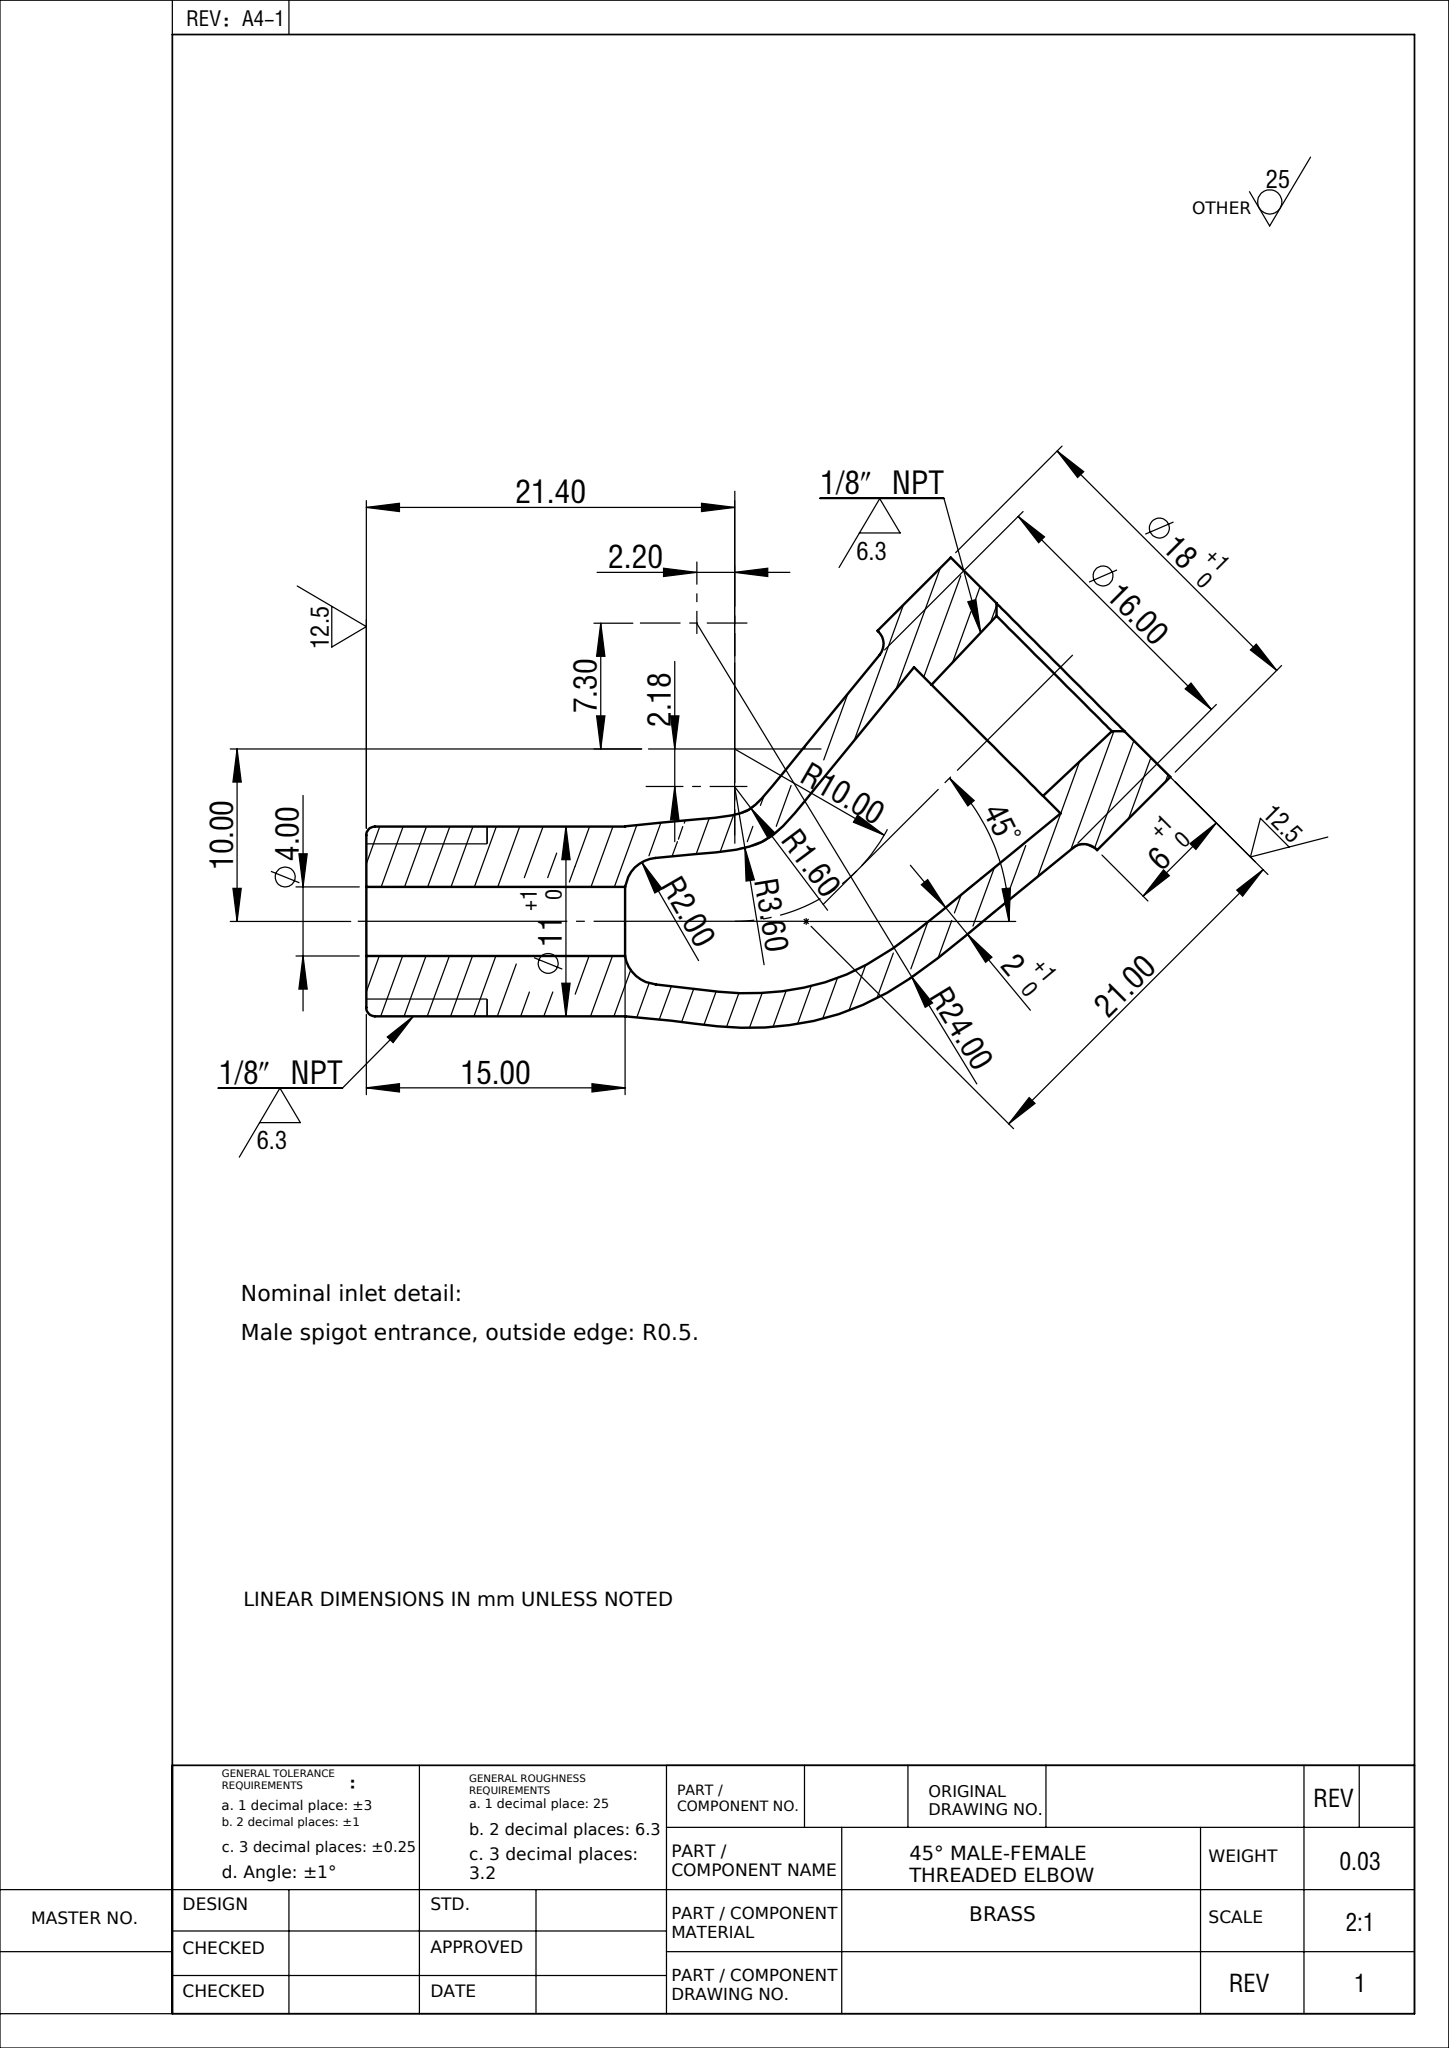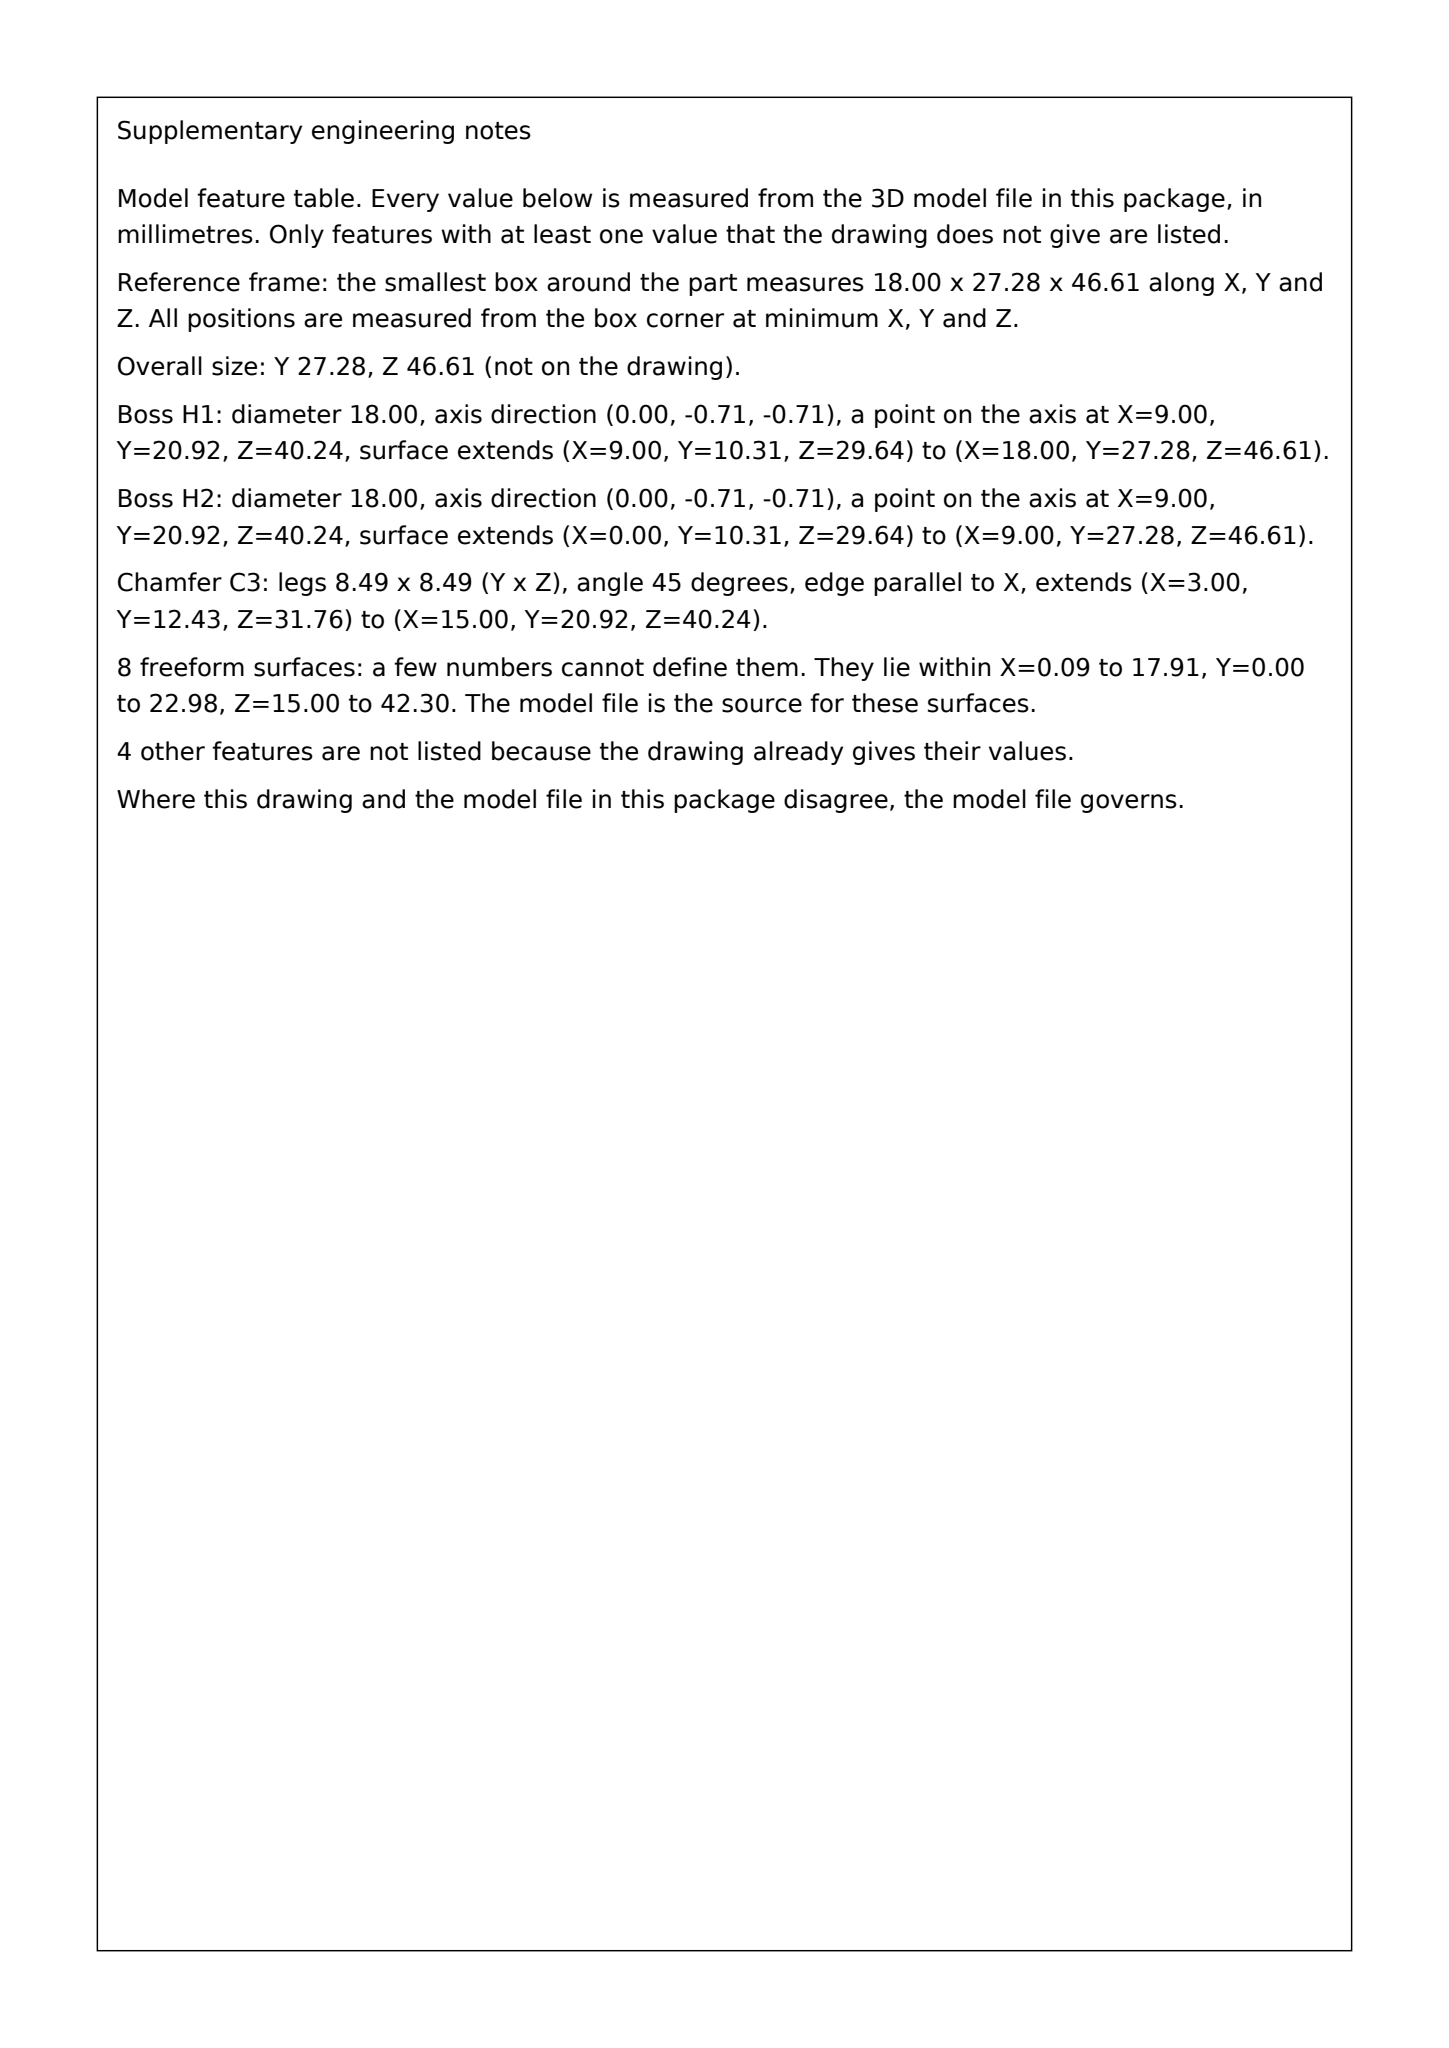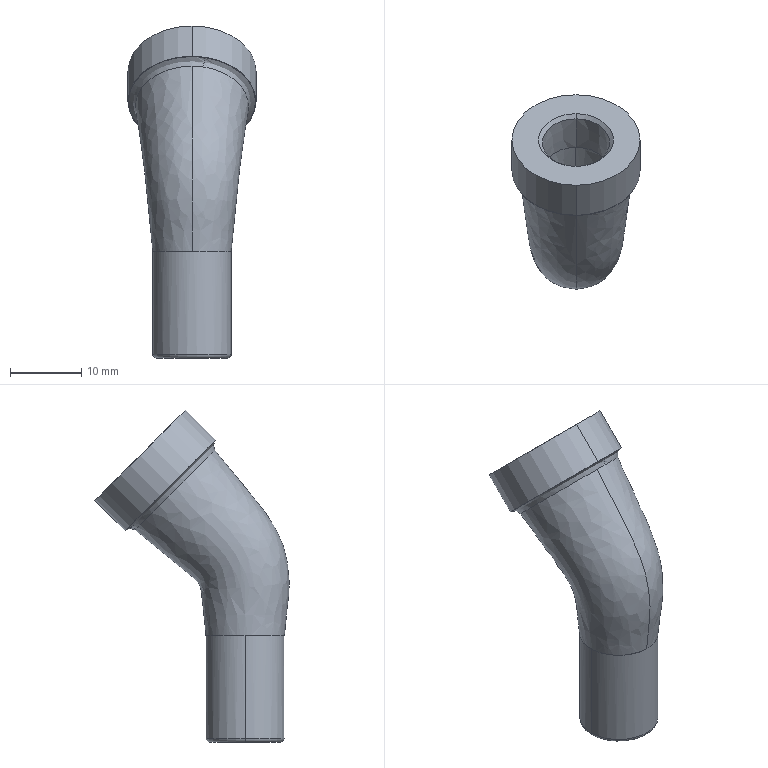Part | SolidWorks | mm | material BRASS | 1 solid | 25 faces | box 18 x 27.28 x 46.61 mm | volume 4182 mm3 | spline 8 | cylinder 6 | plane 5 | cone 4 | torus 2 | commonest cylinder face diameters 4 x2 11 x2 18 x2